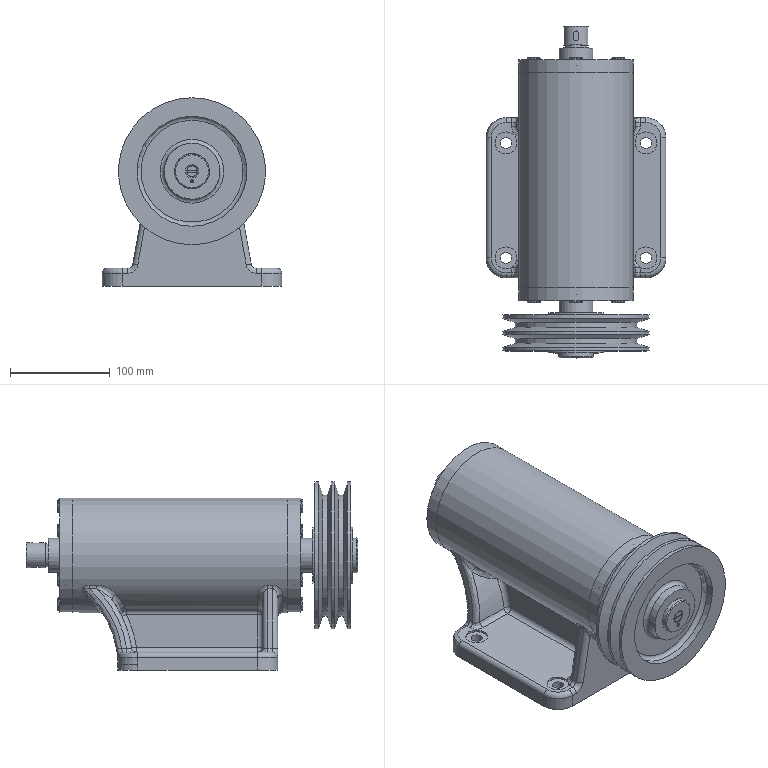Assembly | NX | mm | 26 component files | 52 solids | 750 faces | box 180 x 332 x 188.5 mm | volume 2797000 mm3 | plane 330 | cylinder 191 | cone 142 | torus 52 | spline 27 | sphere 8 | commonest cylinder face diameters 10 x28 11.25 x24 6.619 x12 13 x12 6.8 x12 9 x12 15 x12 35 x9
Bill of materials:
unnamed part 1 | 2 |  | Flat annular ring (washer-like): thin disc with a large concentric through-hole and chamfered outer edges.
GB-T70.1-2000,M8x25 | 12 |  | Hexagon Socket Head Cap Screw, GB-T 70.1-2000,M8x25
unnamed part 2 | 1 |  | Solid elongated block with fully rounded ends (obround/stadium plan shape) and small edge chamfers or rounds on the top and bottom perimeters; resembles a round-ended parallel key.
unnamed part 3 | 1 |  | Circular disc with a central countersunk through-hole, one smaller off-center plain through-hole, and a chamfer on one outer edge.
unnamed part 4 | 2 |  | Circular flange plate with a central through-bore, six through-holes evenly spaced on a bolt circle, and a raised concentric spigot/boss on one face.
unnamed part 5 | 1 |  | Slotted countersunk (flat) head screw-like fastener: conical head with a straight drive slot across the head face, and a plain cylindrical shank.
unnamed part 6 | 1 |  | Thin flat annular ring with a narrow radial wall and rectangular cross-section.
unnamed part 7 | 1 |  | Two-groove V-belt-style pulley/sheave with a central hub boss on both sides and a keyed central bore.
unnamed part 8 | 2 |  | Rolling-element bearing representation: outer ring, inner ring, and a ring of rolling elements between them; inner ring extends axially beyond outer ring on one side.
unnamed part 9 | 1 |  | Housing/bracket with a horizontal hollow cylindrical tube supported on a rectangular base plate by two webs (one straight, one curved); one tube end face has six holes on a circle, and the base has four corner holes.
unnamed part 10 | 1 |  | Solid plain cylindrical pin with chamfered ends on both sides.
unnamed part 11 | 1 |  | Stepped cylindrical shaft with several diameter steps, a larger central section, keyway slots near both ends, and small holes in one end face.
Mates:
1. fix | housing 1 component
2. concentric | key_A_8x7x24 1 edge | shaft 1 edge
3. concentric | bearing_30307 2 edge | shaft 1 edge
4. concentric | end_cap 2 edge | bearing_30307 2 edge
5. concentric | felt_ring 2 edge | end_cap 2 edge
6. concentric | end_cap 2 edge | housing 1 edge
7. concentric | pulley 1 edge | shaft 1 edge
8. concentric | circlip_35 1 edge | pulley 1 edge
9. concentric | pin_3x12 1 edge | circlip_35 1 edge
10. concentric | adjusting_ring 1 edge | end_cap 1 edge
11. concentric | felt_ring 1 edge | end_cap 1 edge
12. concentric | bearing_30307 1 edge | adjusting_ring 1 edge
13. concentric | end_cap 1 edge | housing 1 edge
14. concentric | screw_M6x18 1 edge | circlip_35 1 edge
15. bond | housing 1 component | assembly component
16. bond | screw_M8x25 12 component | assembly component
17. bond | screw_M8x25 11 component | assembly component
18. bond | screw_M8x25 10 component | assembly component
19. bond | screw_M8x25 9 component | assembly component
20. bond | screw_M8x25 8 component | assembly component
21. bond | screw_M8x25 7 component | assembly component
22. bond | screw_M8x25 6 component | assembly component
23. bond | screw_M8x25 5 component | assembly component
24. bond | screw_M8x25 4 component | assembly component
25. bond | screw_M8x25 3 component | assembly component
26. bond | screw_M8x25 2 component | assembly component
27. bond | screw_M8x25 1 component | assembly component
28. circular | assembly datumaxis | assembly cartesiancoordinatesystem | assembly cartesiancoordinatesystem | assembly cartesiancoordinatesystem | assembly cartesiancoordinatesystem | assembly cartesiancoordinatesystem | assembly cartesiancoordinatesystem
29. circular | assembly datumaxis | assembly cartesiancoordinatesystem | assembly cartesiancoordinatesystem | assembly cartesiancoordinatesystem | assembly cartesiancoordinatesystem | assembly cartesiancoordinatesystem | assembly cartesiancoordinatesystem